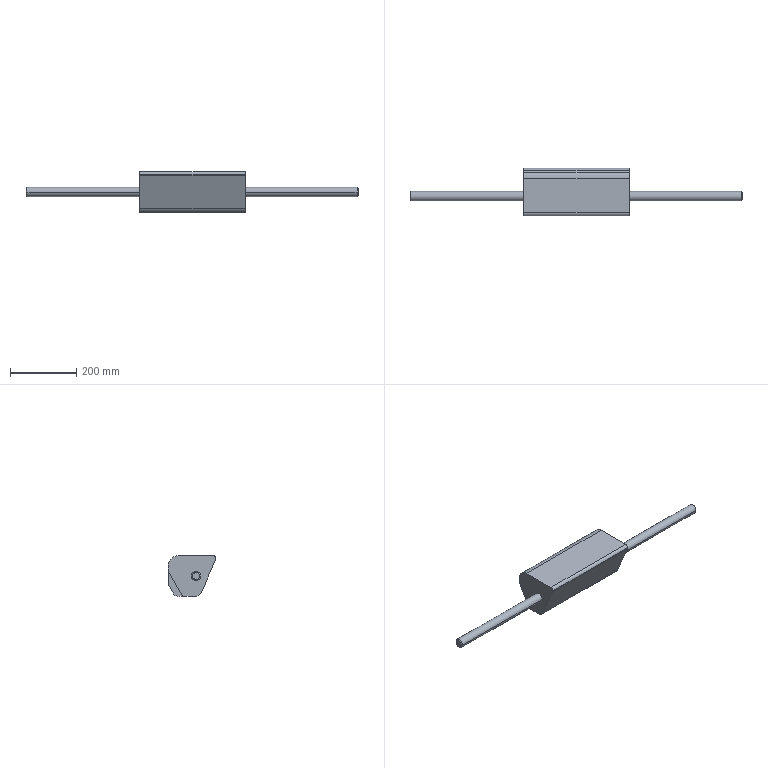Component | SolidWorks | FixedAxis-2 | 1 solid | 28 faces | box 1003 x 143.4 x 123.61 mm | volume 4955800 mm3 | plane 14 | cylinder 10 | cone 4 | commonest cylinder face diameters 28 x4 17.069 x2 73.167 x1 39.953 x1 48 x1 49.516 x1
STEP:
#1=CARTESIAN_POINT('',(-0.09182,31.594,-2.856));
#2=VERTEX_POINT('',#1);
#3=CARTESIAN_POINT('',(-0.09182,32.461,-2.856));
#4=VERTEX_POINT('',#3);
#5=CARTESIAN_POINT('',(-0.09182,32.028,-2.856));
#6=DIRECTION('',(1.,0.,0.));
#7=DIRECTION('',(0.,-1.,0.));
#8=AXIS2_PLACEMENT_3D('',#5,#6,#7);
#9=CIRCLE('',#8,0.4331);
#10=EDGE_CURVE('',#2,#4,#9,.T.);
#11=ORIENTED_EDGE('',*,*,#10,.F.);
#12=CARTESIAN_POINT('',(-0.2099,31.476,-2.856));
#13=VERTEX_POINT('',#12);
#14=CARTESIAN_POINT('',(-0.09182,31.594,-2.856));
#15=DIRECTION('',(-0.7071,-0.7071,-0.));
#16=VECTOR('',#15,39.37);
#17=LINE('',#14,#16);
#18=EDGE_CURVE('',#2,#13,#17,.T.);
#19=ORIENTED_EDGE('',*,*,#18,.T.);
#20=CARTESIAN_POINT('',(-0.2099,32.579,-2.856));
#21=VERTEX_POINT('',#20);
#22=CARTESIAN_POINT('',(-0.2099,32.028,-2.856));
#23=DIRECTION('',(-1.,0.,0.));
#24=DIRECTION('',(0.,-1.,0.));
#25=AXIS2_PLACEMENT_3D('',#22,#23,#24);
#26=CIRCLE('',#25,0.5512);
#27=EDGE_CURVE('',#21,#13,#26,.T.);
#28=ORIENTED_EDGE('',*,*,#27,.F.);
#29=CARTESIAN_POINT('',(-0.09182,32.461,-2.856));
#30=DIRECTION('',(-0.7071,0.7071,0.));
#31=VECTOR('',#30,39.37);
#32=LINE('',#29,#31);
#33=EDGE_CURVE('',#4,#21,#32,.T.);
#34=ORIENTED_EDGE('',*,*,#33,.F.);
#35=EDGE_LOOP('',(#11,#19,#28,#34));
#36=FACE_OUTER_BOUND('',#35,.T.);
#37=CARTESIAN_POINT('',(-0.09182,32.028,-2.856));
#38=DIRECTION('',(-1.,0.,0.));
#39=DIRECTION('',(0.,1.,0.));
#40=AXIS2_PLACEMENT_3D('',#37,#38,#39);
#41=CONICAL_SURFACE('',#40,0.4331,0.7854);
#42=ADVANCED_FACE('',(#36),#41,.T.);
#43=CARTESIAN_POINT('',(-39.58,32.461,-2.856));
#44=VERTEX_POINT('',#43);
#45=CARTESIAN_POINT('',(-39.58,31.594,-2.856));
#46=VERTEX_POINT('',#45);
#47=CARTESIAN_POINT('',(-39.58,32.028,-2.856));
#48=DIRECTION('',(-1.,0.,0.));
#49=DIRECTION('',(0.,1.,0.));
#50=AXIS2_PLACEMENT_3D('',#47,#48,#49);
#51=CIRCLE('',#50,0.4331);
#52=EDGE_CURVE('',#44,#46,#51,.T.);
#53=ORIENTED_EDGE('',*,*,#52,.F.);
#54=CARTESIAN_POINT('',(-39.462,32.579,-2.856));
#55=VERTEX_POINT('',#54);
#56=CARTESIAN_POINT('',(-39.462,32.579,-2.856));
#57=DIRECTION('',(0.7071,0.7071,-0.));
#58=VECTOR('',#57,39.37);
#59=LINE('',#56,#58);
#60=EDGE_CURVE('',#44,#55,#59,.T.);
#61=ORIENTED_EDGE('',*,*,#60,.T.);
#62=CARTESIAN_POINT('',(-39.462,31.476,-2.856));
#63=VERTEX_POINT('',#62);
#64=CARTESIAN_POINT('',(-39.462,32.028,-2.856));
#65=DIRECTION('',(1.,0.,0.));
#66=DIRECTION('',(0.,1.,0.));
#67=AXIS2_PLACEMENT_3D('',#64,#65,#66);
#68=CIRCLE('',#67,0.5512);
#69=EDGE_CURVE('',#63,#55,#68,.T.);
#70=ORIENTED_EDGE('',*,*,#69,.F.);
#71=CARTESIAN_POINT('',(-39.462,31.476,-2.856));
#72=DIRECTION('',(0.7071,-0.7071,0.));
#73=VECTOR('',#72,39.37);
#74=LINE('',#71,#73);
#75=EDGE_CURVE('',#46,#63,#74,.T.);
#76=ORIENTED_EDGE('',*,*,#75,.F.);
#77=EDGE_LOOP('',(#53,#61,#70,#76));
#78=FACE_OUTER_BOUND('',#77,.T.);
#79=CARTESIAN_POINT('',(-39.462,32.028,-2.856));
#80=DIRECTION('',(1.,0.,0.));
#81=DIRECTION('',(0.,-1.,0.));
#82=AXIS2_PLACEMENT_3D('',#79,#80,#81);
#83=CONICAL_SURFACE('',#82,0.5512,0.7854);
#84=ADVANCED_FACE('',(#78),#83,.T.);
#85=CARTESIAN_POINT('',(-13.478,31.476,-2.856));
#86=VERTEX_POINT('',#85);
#87=CARTESIAN_POINT('',(-13.478,32.579,-2.856));
#88=VERTEX_POINT('',#87);
#89=CARTESIAN_POINT('',(-13.478,32.028,-2.856));
#90=DIRECTION('',(1.,0.,0.));
#91=DIRECTION('',(0.,-1.,0.));
#92=AXIS2_PLACEMENT_3D('',#89,#90,#91);
#93=CIRCLE('',#92,0.5512);
#94=EDGE_CURVE('',#86,#88,#93,.T.);
#95=ORIENTED_EDGE('',*,*,#94,.T.);
#96=CARTESIAN_POINT('',(-13.478,32.579,-2.856));
#97=DIRECTION('',(1.,0.,0.));
#98=VECTOR('',#97,39.37);
#99=LINE('',#96,#98);
#100=EDGE_CURVE('',#88,#21,#99,.T.);
#101=ORIENTED_EDGE('',*,*,#100,.T.);
#102=ORIENTED_EDGE('',*,*,#27,.T.);
#103=CARTESIAN_POINT('',(-13.478,31.476,-2.856));
#104=DIRECTION('',(1.,0.,0.));
#105=VECTOR('',#104,39.37);
#106=LINE('',#103,#105);
#107=EDGE_CURVE('',#86,#13,#106,.T.);
#108=ORIENTED_EDGE('',*,*,#107,.F.);
#109=EDGE_LOOP('',(#95,#101,#102,#108));
#110=FACE_OUTER_BOUND('',#109,.T.);
#111=CARTESIAN_POINT('',(-13.478,32.028,-2.856));
#112=DIRECTION('',(1.,0.,0.));
#113=DIRECTION('',(0.,-1.,0.));
#114=AXIS2_PLACEMENT_3D('',#111,#112,#113);
#115=CYLINDRICAL_SURFACE('',#114,0.5512);
#116=ADVANCED_FACE('',(#110),#115,.T.);
#117=ORIENTED_EDGE('',*,*,#69,.T.);
#118=CARTESIAN_POINT('',(-26.076,32.579,-2.856));
#119=VERTEX_POINT('',#118);
#120=CARTESIAN_POINT('',(-39.58,32.579,-2.856));
#121=DIRECTION('',(1.,0.,0.));
#122=VECTOR('',#121,39.37);
#123=LINE('',#120,#122);
#124=EDGE_CURVE('',#55,#119,#123,.T.);
#125=ORIENTED_EDGE('',*,*,#124,.T.);
#126=CARTESIAN_POINT('',(-26.076,31.476,-2.856));
#127=VERTEX_POINT('',#126);
#128=CARTESIAN_POINT('',(-26.076,32.028,-2.856));
#129=DIRECTION('',(1.,0.,0.));
#130=DIRECTION('',(0.,-1.,0.));
#131=AXIS2_PLACEMENT_3D('',#128,#129,#130);
#132=CIRCLE('',#131,0.5512);
#133=EDGE_CURVE('',#127,#119,#132,.T.);
#134=ORIENTED_EDGE('',*,*,#133,.F.);
#135=CARTESIAN_POINT('',(-39.58,31.476,-2.856));
#136=DIRECTION('',(1.,0.,0.));
#137=VECTOR('',#136,39.37);
#138=LINE('',#135,#137);
#139=EDGE_CURVE('',#63,#127,#138,.T.);
#140=ORIENTED_EDGE('',*,*,#139,.F.);
#141=EDGE_LOOP('',(#117,#125,#134,#140));
#142=FACE_OUTER_BOUND('',#141,.T.);
#143=CARTESIAN_POINT('',(-39.58,32.028,-2.856));
#144=DIRECTION('',(1.,0.,0.));
#145=DIRECTION('',(0.,-1.,0.));
#146=AXIS2_PLACEMENT_3D('',#143,#144,#145);
#147=CYLINDRICAL_SURFACE('',#146,0.5512);
#148=ADVANCED_FACE('',(#142),#147,.T.);
#149=CARTESIAN_POINT('',(-26.076,30.025,-0.4232));
#150=VERTEX_POINT('',#149);
#151=CARTESIAN_POINT('',(-26.076,29.689,-0.7592));
#152=VERTEX_POINT('',#151);
#153=CARTESIAN_POINT('',(-26.076,30.025,-0.7592));
#154=DIRECTION('',(1.,0.,0.));
#155=DIRECTION('',(0.,-1.,0.));
#156=AXIS2_PLACEMENT_3D('',#153,#154,#155);
#157=CIRCLE('',#156,0.336);
#158=EDGE_CURVE('',#150,#152,#157,.T.);
#159=ORIENTED_EDGE('',*,*,#158,.T.);
#160=CARTESIAN_POINT('',(-13.478,29.689,-0.7592));
#161=VERTEX_POINT('',#160);
#162=CARTESIAN_POINT('',(-26.076,29.689,-0.7592));
#163=DIRECTION('',(1.,0.,0.));
#164=VECTOR('',#163,39.37);
#165=LINE('',#162,#164);
#166=EDGE_CURVE('',#152,#161,#165,.T.);
#167=ORIENTED_EDGE('',*,*,#166,.T.);
#168=CARTESIAN_POINT('',(-13.478,30.025,-0.4232));
#169=VERTEX_POINT('',#168);
#170=CARTESIAN_POINT('',(-13.478,30.025,-0.7592));
#171=DIRECTION('',(1.,0.,0.));
#172=DIRECTION('',(0.,-1.,0.));
#173=AXIS2_PLACEMENT_3D('',#170,#171,#172);
#174=CIRCLE('',#173,0.336);
#175=EDGE_CURVE('',#169,#161,#174,.T.);
#176=ORIENTED_EDGE('',*,*,#175,.F.);
#177=CARTESIAN_POINT('',(-26.076,30.025,-0.4232));
#178=DIRECTION('',(1.,0.,0.));
#179=VECTOR('',#178,39.37);
#180=LINE('',#177,#179);
#181=EDGE_CURVE('',#150,#169,#180,.T.);
#182=ORIENTED_EDGE('',*,*,#181,.F.);
#183=EDGE_LOOP('',(#159,#167,#176,#182));
#184=FACE_OUTER_BOUND('',#183,.T.);
#185=CARTESIAN_POINT('',(-26.076,30.025,-0.7592));
#186=DIRECTION('',(1.,0.,0.));
#187=DIRECTION('',(0.,-1.,0.));
#188=AXIS2_PLACEMENT_3D('',#185,#186,#187);
#189=CYLINDRICAL_SURFACE('',#188,0.336);
#190=ADVANCED_FACE('',(#184),#189,.T.);
#191=CARTESIAN_POINT('',(-14.304,33.951,-5.29));
#192=VERTEX_POINT('',#191);
#193=CARTESIAN_POINT('',(-14.304,34.617,-5.126));
#194=VERTEX_POINT('',#193);
#195=CARTESIAN_POINT('',(-14.304,33.951,-3.849));
#196=DIRECTION('',(1.,0.,0.));
#197=DIRECTION('',(0.,1.,0.));
#198=AXIS2_PLACEMENT_3D('',#195,#196,#197);
#199=CIRCLE('',#198,1.44);
#200=EDGE_CURVE('',#192,#194,#199,.T.);
#201=ORIENTED_EDGE('',*,*,#200,.F.);
#202=CARTESIAN_POINT('',(-25.249,33.951,-5.29));
#203=VERTEX_POINT('',#202);
#204=CARTESIAN_POINT('',(-26.076,33.951,-5.29));
#205=DIRECTION('',(1.,0.,0.));
#206=VECTOR('',#205,39.37);
#207=LINE('',#204,#206);
#208=EDGE_CURVE('',#203,#192,#207,.T.);
#209=ORIENTED_EDGE('',*,*,#208,.F.);
#210=CARTESIAN_POINT('',(-25.249,34.617,-5.126));
#211=VERTEX_POINT('',#210);
#212=CARTESIAN_POINT('',(-25.249,33.951,-3.849));
#213=DIRECTION('',(1.,0.,0.));
#214=DIRECTION('',(0.,1.,0.));
#215=AXIS2_PLACEMENT_3D('',#212,#213,#214);
#216=CIRCLE('',#215,1.44);
#217=EDGE_CURVE('',#203,#211,#216,.T.);
#218=ORIENTED_EDGE('',*,*,#217,.T.);
#219=CARTESIAN_POINT('',(-26.076,34.617,-5.126));
#220=DIRECTION('',(-1.,0.,0.));
#221=VECTOR('',#220,39.37);
#222=LINE('',#219,#221);
#223=EDGE_CURVE('',#194,#211,#222,.T.);
#224=ORIENTED_EDGE('',*,*,#223,.F.);
#225=EDGE_LOOP('',(#201,#209,#218,#224));
#226=FACE_OUTER_BOUND('',#225,.T.);
#227=CARTESIAN_POINT('',(-26.076,33.951,-3.849));
#228=DIRECTION('',(1.,0.,0.));
#229=DIRECTION('',(0.,-1.,0.));
#230=AXIS2_PLACEMENT_3D('',#227,#228,#229);
#231=CYLINDRICAL_SURFACE('',#230,1.44);
#232=ADVANCED_FACE('',(#226),#231,.T.);
#233=CARTESIAN_POINT('',(-25.249,35.335,-3.887));
#234=VERTEX_POINT('',#233);
#235=CARTESIAN_POINT('',(-14.304,35.335,-3.887));
#236=VERTEX_POINT('',#235);
#237=CARTESIAN_POINT('',(-26.076,35.335,-3.887));
#238=DIRECTION('',(1.,0.,0.));
#239=VECTOR('',#238,39.37);
#240=LINE('',#237,#239);
#241=EDGE_CURVE('',#234,#236,#240,.T.);
#242=ORIENTED_EDGE('',*,*,#241,.T.);
#243=CARTESIAN_POINT('',(-14.304,33.591,-6.898));
#244=DIRECTION('',(0.,-0.501,-0.8654));
#245=VECTOR('',#244,39.37);
#246=LINE('',#243,#245);
#247=EDGE_CURVE('',#236,#194,#246,.T.);
#248=ORIENTED_EDGE('',*,*,#247,.T.);
#249=ORIENTED_EDGE('',*,*,#223,.T.);
#250=CARTESIAN_POINT('',(-25.249,33.591,-6.898));
#251=DIRECTION('',(0.,-0.501,-0.8654));
#252=VECTOR('',#251,39.37);
#253=LINE('',#250,#252);
#254=EDGE_CURVE('',#234,#211,#253,.T.);
#255=ORIENTED_EDGE('',*,*,#254,.F.);
#256=EDGE_LOOP('',(#242,#248,#249,#255));
#257=FACE_OUTER_BOUND('',#256,.T.);
#258=CARTESIAN_POINT('',(-13.478,33.591,-6.898));
#259=DIRECTION('',(0.,-0.8654,0.501));
#260=DIRECTION('',(0.,0.501,0.8654));
#261=AXIS2_PLACEMENT_3D('',#258,#259,#260);
#262=PLANE('',#261);
#263=ADVANCED_FACE('',(#257),#262,.F.);
#264=ORIENTED_EDGE('',*,*,#133,.T.);
#265=CARTESIAN_POINT('',(-26.076,32.028,-2.856));
#266=DIRECTION('',(1.,0.,0.));
#267=DIRECTION('',(0.,-1.,0.));
#268=AXIS2_PLACEMENT_3D('',#265,#266,#267);
#269=CIRCLE('',#268,0.5512);
#270=EDGE_CURVE('',#119,#127,#269,.T.);
#271=ORIENTED_EDGE('',*,*,#270,.T.);
#272=EDGE_LOOP('',(#264,#271));
#273=FACE_BOUND('',#272,.T.);
#274=CARTESIAN_POINT('',(-26.076,35.335,-2.316));
#275=VERTEX_POINT('',#274);
#276=CARTESIAN_POINT('',(-26.076,35.335,-1.602));
#277=VERTEX_POINT('',#276);
#278=CARTESIAN_POINT('',(-26.076,35.335,-4.502));
#279=DIRECTION('',(0.,-0.,1.));
#280=VECTOR('',#279,39.37);
#281=LINE('',#278,#280);
#282=EDGE_CURVE('',#275,#277,#281,.T.);
#283=ORIENTED_EDGE('',*,*,#282,.F.);
#284=CARTESIAN_POINT('',(-26.076,33.613,-5.29));
#285=VERTEX_POINT('',#284);
#286=CARTESIAN_POINT('',(-26.076,34.677,-3.452));
#287=DIRECTION('',(0.,-0.501,-0.8654));
#288=VECTOR('',#287,39.37);
#289=LINE('',#286,#288);
#290=EDGE_CURVE('',#275,#285,#289,.T.);
#291=ORIENTED_EDGE('',*,*,#290,.T.);
#292=CARTESIAN_POINT('',(-26.076,32.104,-5.29));
#293=VERTEX_POINT('',#292);
#294=CARTESIAN_POINT('',(-26.076,31.583,-5.29));
#295=DIRECTION('',(0.,1.,0.));
#296=VECTOR('',#295,39.37);
#297=LINE('',#294,#296);
#298=EDGE_CURVE('',#293,#285,#297,.T.);
#299=ORIENTED_EDGE('',*,*,#298,.F.);
#300=CARTESIAN_POINT('',(-26.076,31.38,-4.81));
#301=VERTEX_POINT('',#300);
#302=CARTESIAN_POINT('',(-26.076,32.104,-4.503));
#303=DIRECTION('',(-1.,0.,0.));
#304=DIRECTION('',(0.,-1.,0.));
#305=AXIS2_PLACEMENT_3D('',#302,#303,#304);
#306=CIRCLE('',#305,0.7865);
#307=EDGE_CURVE('',#293,#301,#306,.T.);
#308=ORIENTED_EDGE('',*,*,#307,.T.);
#309=CARTESIAN_POINT('',(-26.076,29.716,-0.8905));
#310=VERTEX_POINT('',#309);
#311=CARTESIAN_POINT('',(-26.076,29.716,-0.8905));
#312=DIRECTION('',(0.,0.3907,-0.9205));
#313=VECTOR('',#312,39.37);
#314=LINE('',#311,#313);
#315=EDGE_CURVE('',#310,#301,#314,.T.);
#316=ORIENTED_EDGE('',*,*,#315,.F.);
#317=CARTESIAN_POINT('',(-26.076,30.025,-0.7592));
#318=DIRECTION('',(1.,0.,0.));
#319=DIRECTION('',(0.,-1.,0.));
#320=AXIS2_PLACEMENT_3D('',#317,#318,#319);
#321=CIRCLE('',#320,0.336);
#322=EDGE_CURVE('',#152,#310,#321,.T.);
#323=ORIENTED_EDGE('',*,*,#322,.F.);
#324=ORIENTED_EDGE('',*,*,#158,.F.);
#325=CARTESIAN_POINT('',(-26.076,34.143,-0.4232));
#326=VERTEX_POINT('',#325);
#327=CARTESIAN_POINT('',(-26.076,34.547,-0.4232));
#328=DIRECTION('',(0.,-1.,0.));
#329=VECTOR('',#328,39.37);
#330=LINE('',#327,#329);
#331=EDGE_CURVE('',#326,#150,#330,.T.);
#332=ORIENTED_EDGE('',*,*,#331,.F.);
#333=CARTESIAN_POINT('',(-26.076,34.833,-0.7087));
#334=VERTEX_POINT('',#333);
#335=CARTESIAN_POINT('',(-26.076,34.143,-1.398));
#336=DIRECTION('',(-1.,0.,0.));
#337=DIRECTION('',(0.,-1.,0.));
#338=AXIS2_PLACEMENT_3D('',#335,#336,#337);
#339=CIRCLE('',#338,0.9747);
#340=EDGE_CURVE('',#326,#334,#339,.T.);
#341=ORIENTED_EDGE('',*,*,#340,.T.);
#342=CARTESIAN_POINT('',(-26.076,35.058,-0.9338));
#343=VERTEX_POINT('',#342);
#344=CARTESIAN_POINT('',(-26.076,35.335,-1.211));
#345=DIRECTION('',(0.,-0.7071,0.7071));
#346=VECTOR('',#345,39.37);
#347=LINE('',#344,#346);
#348=EDGE_CURVE('',#343,#334,#347,.T.);
#349=ORIENTED_EDGE('',*,*,#348,.F.);
#350=CARTESIAN_POINT('',(-26.076,34.39,-1.602));
#351=DIRECTION('',(-1.,0.,0.));
#352=DIRECTION('',(0.,-1.,-0.));
#353=AXIS2_PLACEMENT_3D('',#350,#351,#352);
#354=CIRCLE('',#353,0.9449);
#355=EDGE_CURVE('',#343,#277,#354,.T.);
#356=ORIENTED_EDGE('',*,*,#355,.T.);
#357=EDGE_LOOP('',(#283,#291,#299,#308,#316,#323,#324,#332,#341,#349,#356));
#358=FACE_OUTER_BOUND('',#357,.T.);
#359=CARTESIAN_POINT('',(-26.076,30.025,-0.7592));
#360=DIRECTION('',(1.,0.,0.));
#361=DIRECTION('',(0.,-1.,0.));
#362=AXIS2_PLACEMENT_3D('',#359,#360,#361);
#363=PLANE('',#362);
#364=ADVANCED_FACE('',(#273,#358),#363,.F.);
#365=CARTESIAN_POINT('',(-13.478,35.335,-2.316));
#366=VERTEX_POINT('',#365);
#367=CARTESIAN_POINT('',(-13.478,33.613,-5.29));
#368=VERTEX_POINT('',#367);
#369=CARTESIAN_POINT('',(-13.478,34.677,-3.452));
#370=DIRECTION('',(0.,-0.501,-0.8654));
#371=VECTOR('',#370,39.37);
#372=LINE('',#369,#371);
#373=EDGE_CURVE('',#366,#368,#372,.T.);
#374=ORIENTED_EDGE('',*,*,#373,.F.);
#375=CARTESIAN_POINT('',(-13.478,35.335,-1.602));
#376=VERTEX_POINT('',#375);
#377=CARTESIAN_POINT('',(-13.478,35.335,-4.502));
#378=DIRECTION('',(0.,-0.,1.));
#379=VECTOR('',#378,39.37);
#380=LINE('',#377,#379);
#381=EDGE_CURVE('',#366,#376,#380,.T.);
#382=ORIENTED_EDGE('',*,*,#381,.T.);
#383=CARTESIAN_POINT('',(-13.478,35.058,-0.9338));
#384=VERTEX_POINT('',#383);
#385=CARTESIAN_POINT('',(-13.478,34.39,-1.602));
#386=DIRECTION('',(1.,0.,0.));
#387=DIRECTION('',(0.,-1.,0.));
#388=AXIS2_PLACEMENT_3D('',#385,#386,#387);
#389=CIRCLE('',#388,0.9449);
#390=EDGE_CURVE('',#376,#384,#389,.T.);
#391=ORIENTED_EDGE('',*,*,#390,.T.);
#392=CARTESIAN_POINT('',(-13.478,34.833,-0.7087));
#393=VERTEX_POINT('',#392);
#394=CARTESIAN_POINT('',(-13.478,35.335,-1.211));
#395=DIRECTION('',(0.,-0.7071,0.7071));
#396=VECTOR('',#395,39.37);
#397=LINE('',#394,#396);
#398=EDGE_CURVE('',#384,#393,#397,.T.);
#399=ORIENTED_EDGE('',*,*,#398,.T.);
#400=CARTESIAN_POINT('',(-13.478,34.143,-0.4232));
#401=VERTEX_POINT('',#400);
#402=CARTESIAN_POINT('',(-13.478,34.143,-1.398));
#403=DIRECTION('',(1.,0.,0.));
#404=DIRECTION('',(0.,-1.,0.));
#405=AXIS2_PLACEMENT_3D('',#402,#403,#404);
#406=CIRCLE('',#405,0.9747);
#407=EDGE_CURVE('',#393,#401,#406,.T.);
#408=ORIENTED_EDGE('',*,*,#407,.T.);
#409=CARTESIAN_POINT('',(-13.478,34.547,-0.4232));
#410=DIRECTION('',(0.,-1.,0.));
#411=VECTOR('',#410,39.37);
#412=LINE('',#409,#411);
#413=EDGE_CURVE('',#401,#169,#412,.T.);
#414=ORIENTED_EDGE('',*,*,#413,.T.);
#415=ORIENTED_EDGE('',*,*,#175,.T.);
#416=CARTESIAN_POINT('',(-13.478,29.716,-0.8905));
#417=VERTEX_POINT('',#416);
#418=CARTESIAN_POINT('',(-13.478,30.025,-0.7592));
#419=DIRECTION('',(1.,0.,0.));
#420=DIRECTION('',(0.,-1.,0.));
#421=AXIS2_PLACEMENT_3D('',#418,#419,#420);
#422=CIRCLE('',#421,0.336);
#423=EDGE_CURVE('',#161,#417,#422,.T.);
#424=ORIENTED_EDGE('',*,*,#423,.T.);
#425=CARTESIAN_POINT('',(-13.478,31.38,-4.81));
#426=VERTEX_POINT('',#425);
#427=CARTESIAN_POINT('',(-13.478,29.716,-0.8905));
#428=DIRECTION('',(0.,0.3907,-0.9205));
#429=VECTOR('',#428,39.37);
#430=LINE('',#427,#429);
#431=EDGE_CURVE('',#417,#426,#430,.T.);
#432=ORIENTED_EDGE('',*,*,#431,.T.);
#433=CARTESIAN_POINT('',(-13.478,32.104,-5.29));
#434=VERTEX_POINT('',#433);
#435=CARTESIAN_POINT('',(-13.478,32.104,-4.503));
#436=DIRECTION('',(1.,0.,0.));
#437=DIRECTION('',(0.,-1.,0.));
#438=AXIS2_PLACEMENT_3D('',#435,#436,#437);
#439=CIRCLE('',#438,0.7865);
#440=EDGE_CURVE('',#426,#434,#439,.T.);
#441=ORIENTED_EDGE('',*,*,#440,.T.);
#442=CARTESIAN_POINT('',(-13.478,31.583,-5.29));
#443=DIRECTION('',(0.,1.,0.));
#444=VECTOR('',#443,39.37);
#445=LINE('',#442,#444);
#446=EDGE_CURVE('',#434,#368,#445,.T.);
#447=ORIENTED_EDGE('',*,*,#446,.T.);
#448=EDGE_LOOP('',(#374,#382,#391,#399,#408,#414,#415,#424,#432,#441,#447));
#449=FACE_OUTER_BOUND('',#448,.T.);
#450=ORIENTED_EDGE('',*,*,#94,.F.);
#451=CARTESIAN_POINT('',(-13.478,32.028,-2.856));
#452=DIRECTION('',(1.,0.,0.));
#453=DIRECTION('',(0.,-1.,0.));
#454=AXIS2_PLACEMENT_3D('',#451,#452,#453);
#455=CIRCLE('',#454,0.5512);
#456=EDGE_CURVE('',#88,#86,#455,.T.);
#457=ORIENTED_EDGE('',*,*,#456,.F.);
#458=EDGE_LOOP('',(#450,#457));
#459=FACE_BOUND('',#458,.T.);
#460=CARTESIAN_POINT('',(-13.478,30.025,-0.7592));
#461=DIRECTION('',(1.,0.,0.));
#462=DIRECTION('',(0.,-1.,0.));
#463=AXIS2_PLACEMENT_3D('',#460,#461,#462);
#464=PLANE('',#463);
#465=ADVANCED_FACE('',(#449,#459),#464,.T.);
#466=CARTESIAN_POINT('',(-14.304,35.335,-2.316));
#467=VERTEX_POINT('',#466);
#468=CARTESIAN_POINT('',(-26.076,35.335,-2.316));
#469=DIRECTION('',(1.,0.,0.));
#470=VECTOR('',#469,39.37);
#471=LINE('',#468,#470);
#472=EDGE_CURVE('',#467,#366,#471,.T.);
#473=ORIENTED_EDGE('',*,*,#472,.F.);
#474=CARTESIAN_POINT('',(-14.304,35.335,-4.502));
#475=DIRECTION('',(0.,-0.,1.));
#476=VECTOR('',#475,39.37);
#477=LINE('',#474,#476);
#478=EDGE_CURVE('',#236,#467,#477,.T.);
#479=ORIENTED_EDGE('',*,*,#478,.F.);
#480=ORIENTED_EDGE('',*,*,#241,.F.);
#481=CARTESIAN_POINT('',(-25.249,35.335,-2.316));
#482=VERTEX_POINT('',#481);
#483=CARTESIAN_POINT('',(-25.249,35.335,-4.502));
#484=DIRECTION('',(0.,-0.,1.));
#485=VECTOR('',#484,39.37);
#486=LINE('',#483,#485);
#487=EDGE_CURVE('',#234,#482,#486,.T.);
#488=ORIENTED_EDGE('',*,*,#487,.T.);
#489=CARTESIAN_POINT('',(-26.076,35.335,-2.316));
#490=DIRECTION('',(1.,0.,0.));
#491=VECTOR('',#490,39.37);
#492=LINE('',#489,#491);
#493=EDGE_CURVE('',#275,#482,#492,.T.);
#494=ORIENTED_EDGE('',*,*,#493,.F.);
#495=ORIENTED_EDGE('',*,*,#282,.T.);
#496=CARTESIAN_POINT('',(-26.076,35.335,-1.602));
#497=DIRECTION('',(1.,0.,0.));
#498=VECTOR('',#497,39.37);
#499=LINE('',#496,#498);
#500=EDGE_CURVE('',#277,#376,#499,.T.);
#501=ORIENTED_EDGE('',*,*,#500,.T.);
#502=ORIENTED_EDGE('',*,*,#381,.F.);
#503=EDGE_LOOP('',(#473,#479,#480,#488,#494,#495,#501,#502));
#504=FACE_OUTER_BOUND('',#503,.T.);
#505=CARTESIAN_POINT('',(-26.076,35.335,-4.502));
#506=DIRECTION('',(0.,1.,0.));
#507=DIRECTION('',(0.,0.,-1.));
#508=AXIS2_PLACEMENT_3D('',#505,#506,#507);
#509=PLANE('',#508);
#510=ADVANCED_FACE('',(#504),#509,.T.);
#511=CARTESIAN_POINT('',(-14.304,33.613,-5.29));
#512=VERTEX_POINT('',#511);
#513=CARTESIAN_POINT('',(-26.076,33.613,-5.29));
#514=DIRECTION('',(-1.,0.,0.));
#515=VECTOR('',#514,39.37);
#516=LINE('',#513,#515);
#517=EDGE_CURVE('',#368,#512,#516,.T.);
#518=ORIENTED_EDGE('',*,*,#517,.F.);
#519=ORIENTED_EDGE('',*,*,#446,.F.);
#520=CARTESIAN_POINT('',(-26.076,32.104,-5.29));
#521=DIRECTION('',(-1.,0.,0.));
#522=VECTOR('',#521,39.37);
#523=LINE('',#520,#522);
#524=EDGE_CURVE('',#434,#293,#523,.T.);
#525=ORIENTED_EDGE('',*,*,#524,.T.);
#526=ORIENTED_EDGE('',*,*,#298,.T.);
#527=CARTESIAN_POINT('',(-25.249,33.613,-5.29));
#528=VERTEX_POINT('',#527);
#529=CARTESIAN_POINT('',(-26.076,33.613,-5.29));
#530=DIRECTION('',(-1.,0.,0.));
#531=VECTOR('',#530,39.37);
#532=LINE('',#529,#531);
#533=EDGE_CURVE('',#528,#285,#532,.T.);
#534=ORIENTED_EDGE('',*,*,#533,.F.);
#535=CARTESIAN_POINT('',(-25.249,31.583,-5.29));
#536=DIRECTION('',(0.,1.,0.));
#537=VECTOR('',#536,39.37);
#538=LINE('',#535,#537);
#539=EDGE_CURVE('',#528,#203,#538,.T.);
#540=ORIENTED_EDGE('',*,*,#539,.T.);
#541=ORIENTED_EDGE('',*,*,#208,.T.);
#542=CARTESIAN_POINT('',(-14.304,31.583,-5.29));
#543=DIRECTION('',(0.,1.,0.));
#544=VECTOR('',#543,39.37);
#545=LINE('',#542,#544);
#546=EDGE_CURVE('',#512,#192,#545,.T.);
#547=ORIENTED_EDGE('',*,*,#546,.F.);
#548=EDGE_LOOP('',(#518,#519,#525,#526,#534,#540,#541,#547));
#549=FACE_OUTER_BOUND('',#548,.T.);
#550=CARTESIAN_POINT('',(-26.076,31.583,-5.29));
#551=DIRECTION('',(0.,0.,-1.));
#552=DIRECTION('',(-1.,0.,0.));
#553=AXIS2_PLACEMENT_3D('',#550,#551,#552);
#554=PLANE('',#553);
#555=ADVANCED_FACE('',(#549),#554,.T.);
#556=ORIENTED_EDGE('',*,*,#315,.T.);
#557=CARTESIAN_POINT('',(-26.076,31.38,-4.81));
#558=DIRECTION('',(1.,0.,0.));
#559=VECTOR('',#558,39.37);
#560=LINE('',#557,#559);
#561=EDGE_CURVE('',#301,#426,#560,.T.);
#562=ORIENTED_EDGE('',*,*,#561,.T.);
#563=ORIENTED_EDGE('',*,*,#431,.F.);
#564=CARTESIAN_POINT('',(-26.076,29.716,-0.8905));
#565=DIRECTION('',(1.,0.,0.));
#566=VECTOR('',#565,39.37);
#567=LINE('',#564,#566);
#568=EDGE_CURVE('',#310,#417,#567,.T.);
#569=ORIENTED_EDGE('',*,*,#568,.F.);
#570=EDGE_LOOP('',(#556,#562,#563,#569));
#571=FACE_OUTER_BOUND('',#570,.T.);
#572=CARTESIAN_POINT('',(-26.076,29.716,-0.8905));
#573=DIRECTION('',(0.,-0.9205,-0.3907));
#574=DIRECTION('',(0.,-0.3907,0.9205));
#575=AXIS2_PLACEMENT_3D('',#572,#573,#574);
#576=PLANE('',#575);
#577=ADVANCED_FACE('',(#571),#576,.T.);
#578=ORIENTED_EDGE('',*,*,#166,.F.);
#579=ORIENTED_EDGE('',*,*,#322,.T.);
#580=ORIENTED_EDGE('',*,*,#568,.T.);
#581=ORIENTED_EDGE('',*,*,#423,.F.);
#582=EDGE_LOOP('',(#578,#579,#580,#581));
#583=FACE_OUTER_BOUND('',#582,.T.);
#584=CARTESIAN_POINT('',(-26.076,30.025,-0.7592));
#585=DIRECTION('',(1.,0.,0.));
#586=DIRECTION('',(0.,-1.,0.));
#587=AXIS2_PLACEMENT_3D('',#584,#585,#586);
#588=CYLINDRICAL_SURFACE('',#587,0.336);
#589=ADVANCED_FACE('',(#583),#588,.T.);
#590=ORIENTED_EDGE('',*,*,#413,.F.);
#591=CARTESIAN_POINT('',(-26.076,34.143,-0.4232));
#592=DIRECTION('',(-1.,0.,0.));
#593=VECTOR('',#592,39.37);
#594=LINE('',#591,#593);
#595=EDGE_CURVE('',#401,#326,#594,.T.);
#596=ORIENTED_EDGE('',*,*,#595,.T.);
#597=ORIENTED_EDGE('',*,*,#331,.T.);
#598=ORIENTED_EDGE('',*,*,#181,.T.);
#599=EDGE_LOOP('',(#590,#596,#597,#598));
#600=FACE_OUTER_BOUND('',#599,.T.);
#601=CARTESIAN_POINT('',(-26.076,34.547,-0.4232));
#602=DIRECTION('',(0.,0.,1.));
#603=DIRECTION('',(1.,0.,0.));
#604=AXIS2_PLACEMENT_3D('',#601,#602,#603);
#605=PLANE('',#604);
#606=ADVANCED_FACE('',(#600),#605,.T.);
#607=ORIENTED_EDGE('',*,*,#348,.T.);
#608=CARTESIAN_POINT('',(-26.076,34.833,-0.7087));
#609=DIRECTION('',(1.,0.,0.));
#610=VECTOR('',#609,39.37);
#611=LINE('',#608,#610);
#612=EDGE_CURVE('',#334,#393,#611,.T.);
#613=ORIENTED_EDGE('',*,*,#612,.T.);
#614=ORIENTED_EDGE('',*,*,#398,.F.);
#615=CARTESIAN_POINT('',(-26.076,35.058,-0.9338));
#616=DIRECTION('',(-1.,0.,0.));
#617=VECTOR('',#616,39.37);
#618=LINE('',#615,#617);
#619=EDGE_CURVE('',#384,#343,#618,.T.);
#620=ORIENTED_EDGE('',*,*,#619,.T.);
#621=EDGE_LOOP('',(#607,#613,#614,#620));
#622=FACE_OUTER_BOUND('',#621,.T.);
#623=CARTESIAN_POINT('',(-26.076,35.335,-1.211));
#624=DIRECTION('',(0.,0.7071,0.7071));
#625=DIRECTION('',(0.,0.7071,-0.7071));
#626=AXIS2_PLACEMENT_3D('',#623,#624,#625);
#627=PLANE('',#626);
#628=ADVANCED_FACE('',(#622),#627,.T.);
#629=ORIENTED_EDGE('',*,*,#124,.F.);
#630=CARTESIAN_POINT('',(-39.462,32.028,-2.856));
#631=DIRECTION('',(1.,0.,0.));
#632=DIRECTION('',(0.,1.,0.));
#633=AXIS2_PLACEMENT_3D('',#630,#631,#632);
#634=CIRCLE('',#633,0.5512);
#635=EDGE_CURVE('',#55,#63,#634,.T.);
#636=ORIENTED_EDGE('',*,*,#635,.T.);
#637=ORIENTED_EDGE('',*,*,#139,.T.);
#638=ORIENTED_EDGE('',*,*,#270,.F.);
#639=EDGE_LOOP('',(#629,#636,#637,#638));
#640=FACE_OUTER_BOUND('',#639,.T.);
#641=CARTESIAN_POINT('',(-39.58,32.028,-2.856));
#642=DIRECTION('',(1.,0.,0.));
#643=DIRECTION('',(0.,-1.,0.));
#644=AXIS2_PLACEMENT_3D('',#641,#642,#643);
#645=CYLINDRICAL_SURFACE('',#644,0.5512);
#646=ADVANCED_FACE('',(#640),#645,.T.);
#647=CARTESIAN_POINT('',(-39.58,32.028,-2.856));
#648=DIRECTION('',(-1.,0.,0.));
#649=DIRECTION('',(0.,1.,0.));
#650=AXIS2_PLACEMENT_3D('',#647,#648,#649);
#651=CIRCLE('',#650,0.4331);
#652=EDGE_CURVE('',#46,#44,#651,.T.);
#653=ORIENTED_EDGE('',*,*,#652,.T.);
#654=ORIENTED_EDGE('',*,*,#52,.T.);
#655=EDGE_LOOP('',(#653,#654));
#656=FACE_OUTER_BOUND('',#655,.T.);
#657=CARTESIAN_POINT('',(-39.58,32.579,-2.856));
#658=DIRECTION('',(-1.,0.,0.));
#659=DIRECTION('',(0.,1.,0.));
#660=AXIS2_PLACEMENT_3D('',#657,#658,#659);
#661=PLANE('',#660);
#662=ADVANCED_FACE('',(#656),#661,.T.);
#663=ORIENTED_EDGE('',*,*,#100,.F.);
#664=ORIENTED_EDGE('',*,*,#456,.T.);
#665=ORIENTED_EDGE('',*,*,#107,.T.);
#666=CARTESIAN_POINT('',(-0.2099,32.028,-2.856));
#667=DIRECTION('',(-1.,0.,0.));
#668=DIRECTION('',(0.,-1.,0.));
#669=AXIS2_PLACEMENT_3D('',#666,#667,#668);
#670=CIRCLE('',#669,0.5512);
#671=EDGE_CURVE('',#13,#21,#670,.T.);
#672=ORIENTED_EDGE('',*,*,#671,.T.);
#673=EDGE_LOOP('',(#663,#664,#665,#672));
#674=FACE_OUTER_BOUND('',#673,.T.);
#675=CARTESIAN_POINT('',(-13.478,32.028,-2.856));
#676=DIRECTION('',(1.,0.,0.));
#677=DIRECTION('',(0.,-1.,0.));
#678=AXIS2_PLACEMENT_3D('',#675,#676,#677);
#679=CYLINDRICAL_SURFACE('',#678,0.5512);
#680=ADVANCED_FACE('',(#674),#679,.T.);
#681=CARTESIAN_POINT('',(-0.09182,32.028,-2.856));
#682=DIRECTION('',(1.,0.,0.));
#683=DIRECTION('',(0.,-1.,0.));
#684=AXIS2_PLACEMENT_3D('',#681,#682,#683);
#685=CIRCLE('',#684,0.4331);
#686=EDGE_CURVE('',#4,#2,#685,.T.);
#687=ORIENTED_EDGE('',*,*,#686,.T.);
#688=ORIENTED_EDGE('',*,*,#10,.T.);
#689=EDGE_LOOP('',(#687,#688));
#690=FACE_OUTER_BOUND('',#689,.T.);
#691=CARTESIAN_POINT('',(-0.09182,32.028,-2.856));
#692=DIRECTION('',(1.,0.,0.));
#693=DIRECTION('',(0.,-1.,0.));
#694=AXIS2_PLACEMENT_3D('',#691,#692,#693);
#695=PLANE('',#694);
#696=ADVANCED_FACE('',(#690),#695,.T.);
#697=ORIENTED_EDGE('',*,*,#60,.F.);
#698=ORIENTED_EDGE('',*,*,#652,.F.);
#699=ORIENTED_EDGE('',*,*,#75,.T.);
#700=ORIENTED_EDGE('',*,*,#635,.F.);
#701=EDGE_LOOP('',(#697,#698,#699,#700));
#702=FACE_OUTER_BOUND('',#701,.T.);
#703=CARTESIAN_POINT('',(-39.462,32.028,-2.856));
#704=DIRECTION('',(1.,0.,0.));
#705=DIRECTION('',(0.,-1.,0.));
#706=AXIS2_PLACEMENT_3D('',#703,#704,#705);
#707=CONICAL_SURFACE('',#706,0.5512,0.7854);
#708=ADVANCED_FACE('',(#702),#707,.T.);
#709=ORIENTED_EDGE('',*,*,#18,.F.);
#710=ORIENTED_EDGE('',*,*,#686,.F.);
#711=ORIENTED_EDGE('',*,*,#33,.T.);
#712=ORIENTED_EDGE('',*,*,#671,.F.);
#713=EDGE_LOOP('',(#709,#710,#711,#712));
#714=FACE_OUTER_BOUND('',#713,.T.);
#715=CARTESIAN_POINT('',(-0.09182,32.028,-2.856));
#716=DIRECTION('',(-1.,0.,0.));
#717=DIRECTION('',(0.,1.,0.));
#718=AXIS2_PLACEMENT_3D('',#715,#716,#717);
#719=CONICAL_SURFACE('',#718,0.4331,0.7854);
#720=ADVANCED_FACE('',(#714),#719,.T.);
#721=ORIENTED_EDGE('',*,*,#307,.F.);
#722=ORIENTED_EDGE('',*,*,#524,.F.);
#723=ORIENTED_EDGE('',*,*,#440,.F.);
#724=ORIENTED_EDGE('',*,*,#561,.F.);
#725=EDGE_LOOP('',(#721,#722,#723,#724));
#726=FACE_OUTER_BOUND('',#725,.T.);
#727=CARTESIAN_POINT('',(-26.076,32.104,-4.503));
#728=DIRECTION('',(1.,0.,0.));
#729=DIRECTION('',(0.,-1.,0.));
#730=AXIS2_PLACEMENT_3D('',#727,#728,#729);
#731=CYLINDRICAL_SURFACE('',#730,0.7865);
#732=ADVANCED_FACE('',(#726),#731,.T.);
#733=ORIENTED_EDGE('',*,*,#355,.F.);
#734=ORIENTED_EDGE('',*,*,#619,.F.);
#735=ORIENTED_EDGE('',*,*,#390,.F.);
#736=ORIENTED_EDGE('',*,*,#500,.F.);
#737=EDGE_LOOP('',(#733,#734,#735,#736));
#738=FACE_OUTER_BOUND('',#737,.T.);
#739=CARTESIAN_POINT('',(-26.076,34.39,-1.602));
#740=DIRECTION('',(1.,0.,0.));
#741=DIRECTION('',(0.,-1.,0.));
#742=AXIS2_PLACEMENT_3D('',#739,#740,#741);
#743=CYLINDRICAL_SURFACE('',#742,0.9449);
#744=ADVANCED_FACE('',(#738),#743,.T.);
#745=ORIENTED_EDGE('',*,*,#340,.F.);
#746=ORIENTED_EDGE('',*,*,#595,.F.);
#747=ORIENTED_EDGE('',*,*,#407,.F.);
#748=ORIENTED_EDGE('',*,*,#612,.F.);
#749=EDGE_LOOP('',(#745,#746,#747,#748));
#750=FACE_OUTER_BOUND('',#749,.T.);
#751=CARTESIAN_POINT('',(-26.076,34.143,-1.398));
#752=DIRECTION('',(1.,0.,0.));
#753=DIRECTION('',(0.,-1.,0.));
#754=AXIS2_PLACEMENT_3D('',#751,#752,#753);
#755=CYLINDRICAL_SURFACE('',#754,0.9747);
#756=ADVANCED_FACE('',(#750),#755,.T.);
#757=ORIENTED_EDGE('',*,*,#493,.T.);
#758=CARTESIAN_POINT('',(-25.249,32.91,-6.504));
#759=DIRECTION('',(0.,0.501,0.8654));
#760=VECTOR('',#759,39.37);
#761=LINE('',#758,#760);
#762=EDGE_CURVE('',#528,#482,#761,.T.);
#763=ORIENTED_EDGE('',*,*,#762,.F.);
#764=ORIENTED_EDGE('',*,*,#533,.T.);
#765=ORIENTED_EDGE('',*,*,#290,.F.);
#766=EDGE_LOOP('',(#757,#763,#764,#765));
#767=FACE_OUTER_BOUND('',#766,.T.);
#768=CARTESIAN_POINT('',(-25.249,32.91,-6.504));
#769=DIRECTION('',(0.,-0.8654,0.501));
#770=DIRECTION('',(0.,0.501,0.8654));
#771=AXIS2_PLACEMENT_3D('',#768,#769,#770);
#772=PLANE('',#771);
#773=ADVANCED_FACE('',(#767),#772,.F.);
#774=ORIENTED_EDGE('',*,*,#254,.T.);
#775=ORIENTED_EDGE('',*,*,#217,.F.);
#776=ORIENTED_EDGE('',*,*,#539,.F.);
#777=ORIENTED_EDGE('',*,*,#762,.T.);
#778=ORIENTED_EDGE('',*,*,#487,.F.);
#779=EDGE_LOOP('',(#774,#775,#776,#777,#778));
#780=FACE_OUTER_BOUND('',#779,.T.);
#781=CARTESIAN_POINT('',(-25.249,32.028,-2.856));
#782=DIRECTION('',(-1.,0.,0.));
#783=DIRECTION('',(0.,1.,0.));
#784=AXIS2_PLACEMENT_3D('',#781,#782,#783);
#785=PLANE('',#784);
#786=ADVANCED_FACE('',(#780),#785,.T.);
#787=ORIENTED_EDGE('',*,*,#472,.T.);
#788=ORIENTED_EDGE('',*,*,#373,.T.);
#789=ORIENTED_EDGE('',*,*,#517,.T.);
#790=CARTESIAN_POINT('',(-14.304,32.91,-6.504));
#791=DIRECTION('',(0.,0.501,0.8654));
#792=VECTOR('',#791,39.37);
#793=LINE('',#790,#792);
#794=EDGE_CURVE('',#512,#467,#793,.T.);
#795=ORIENTED_EDGE('',*,*,#794,.T.);
#796=EDGE_LOOP('',(#787,#788,#789,#795));
#797=FACE_OUTER_BOUND('',#796,.T.);
#798=CARTESIAN_POINT('',(-13.438,32.91,-6.504));
#799=DIRECTION('',(0.,-0.8654,0.501));
#800=DIRECTION('',(0.,0.501,0.8654));
#801=AXIS2_PLACEMENT_3D('',#798,#799,#800);
#802=PLANE('',#801);
#803=ADVANCED_FACE('',(#797),#802,.F.);
#804=ORIENTED_EDGE('',*,*,#478,.T.);
#805=ORIENTED_EDGE('',*,*,#794,.F.);
#806=ORIENTED_EDGE('',*,*,#546,.T.);
#807=ORIENTED_EDGE('',*,*,#200,.T.);
#808=ORIENTED_EDGE('',*,*,#247,.F.);
#809=EDGE_LOOP('',(#804,#805,#806,#807,#808));
#810=FACE_OUTER_BOUND('',#809,.T.);
#811=CARTESIAN_POINT('',(-14.304,32.028,-2.856));
#812=DIRECTION('',(-1.,0.,0.));
#813=DIRECTION('',(0.,1.,0.));
#814=AXIS2_PLACEMENT_3D('',#811,#812,#813);
#815=PLANE('',#814);
#816=ADVANCED_FACE('',(#810),#815,.F.);
#817=CLOSED_SHELL('',(#42,#84,#116,#148,#190,#232,#263,#364,#465,#510,#555,#577,#589,#606,#628,#646,#662,#680,#696,#708,#720,#732,#744,#756,#773,#786,#803,#816));
#818=MANIFOLD_SOLID_BREP('',#817);
#819=CARTESIAN_POINT('',(0.,0.,0.));
#820=DIRECTION('',(0.,0.,1.));
#821=DIRECTION('',(1.,0.,0.));
#822=AXIS2_PLACEMENT_3D('',#819,#820,#821);
#823=(LENGTH_UNIT()NAMED_UNIT(*)SI_UNIT($,.METRE.));
#824=LENGTH_MEASURE_WITH_UNIT(LENGTH_MEASURE(0.0254),#823);
#825=DIMENSIONAL_EXPONENTS(1.,0.,0.,0.,0.,0.,0.);
#826=(CONVERSION_BASED_UNIT('',#824)LENGTH_UNIT()NAMED_UNIT(#825));
#827=UNCERTAINTY_MEASURE_WITH_UNIT(LENGTH_MEASURE(0.00001),#826,'','');
#828=(NAMED_UNIT(*)PLANE_ANGLE_UNIT()SI_UNIT($,.RADIAN.));
#829=(NAMED_UNIT(*)SI_UNIT($,.STERADIAN.)SOLID_ANGLE_UNIT());
#830=(GEOMETRIC_REPRESENTATION_CONTEXT(3)GLOBAL_UNCERTAINTY_ASSIGNED_CONTEXT((#827))GLOBAL_UNIT_ASSIGNED_CONTEXT((#826,#828,#829))REPRESENTATION_CONTEXT('',''));
#831=ADVANCED_BREP_SHAPE_REPRESENTATION('',(#818,#822),#830);
#832=COLOUR_RGB('',0.7922,0.8196,0.9333);
#833=FILL_AREA_STYLE_COLOUR('',#832);
#834=FILL_AREA_STYLE('',(#833));
#835=SURFACE_STYLE_FILL_AREA(#834);
#836=SURFACE_SIDE_STYLE('',(#835));
#837=SURFACE_STYLE_USAGE(.BOTH.,#836);
#838=PRESENTATION_STYLE_ASSIGNMENT((#837));
#839=STYLED_ITEM('',(#838),#818);
#840=(LENGTH_UNIT()NAMED_UNIT(*)SI_UNIT($,.METRE.));
#841=LENGTH_MEASURE_WITH_UNIT(LENGTH_MEASURE(0.0254),#840);
#842=DIMENSIONAL_EXPONENTS(1.,0.,0.,0.,0.,0.,0.);
#843=(CONVERSION_BASED_UNIT('',#841)LENGTH_UNIT()NAMED_UNIT(#842));
#844=UNCERTAINTY_MEASURE_WITH_UNIT(LENGTH_MEASURE(0.00001),#843,'','');
#845=(NAMED_UNIT(*)PLANE_ANGLE_UNIT()SI_UNIT($,.RADIAN.));
#846=(NAMED_UNIT(*)SI_UNIT($,.STERADIAN.)SOLID_ANGLE_UNIT());
#847=(GEOMETRIC_REPRESENTATION_CONTEXT(3)GLOBAL_UNCERTAINTY_ASSIGNED_CONTEXT((#844))GLOBAL_UNIT_ASSIGNED_CONTEXT((#843,#845,#846))REPRESENTATION_CONTEXT('',''));
#848=MECHANICAL_DESIGN_GEOMETRIC_PRESENTATION_REPRESENTATION('',(#839),#847);
#849=PRESENTATION_LAYER_ASSIGNMENT('','',(#839));